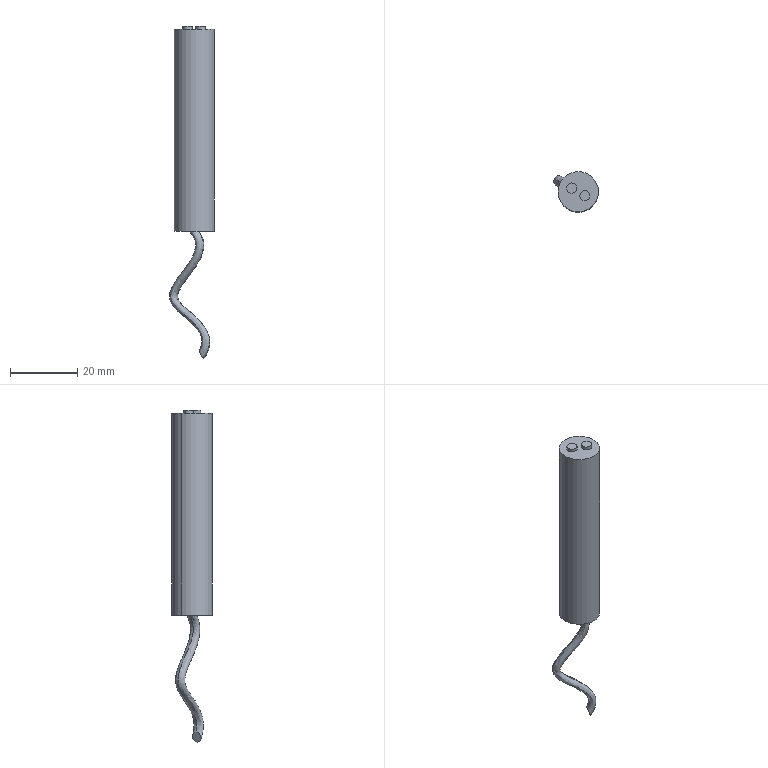Component | SolidWorks | 04_12PhotoelectricSwitch-3 | 1 solid | 13 faces | box 13.38 x 12 x 98.73 mm | volume 7034 mm3 | cylinder 6 | plane 5 | spline 2 | commonest cylinder face diameters 3 x4 12 x2
STEP:
#1=CARTESIAN_POINT('',(3.235,-4.292,15.551));
#2=VERTEX_POINT('',#1);
#3=CARTESIAN_POINT('',(3.133,-4.233,15.551));
#4=VERTEX_POINT('',#3);
#5=CARTESIAN_POINT('',(3.184,-4.263,15.551));
#6=DIRECTION('',(-0.,0.,1.));
#7=DIRECTION('',(-0.8652,0.5014,0.));
#8=AXIS2_PLACEMENT_3D('',#5,#6,#7);
#9=CIRCLE('',#8,0.05906);
#10=EDGE_CURVE('',#2,#4,#9,.T.);
#11=ORIENTED_EDGE('',*,*,#10,.F.);
#12=CARTESIAN_POINT('',(3.235,-4.292,15.512));
#13=VERTEX_POINT('',#12);
#14=CARTESIAN_POINT('',(3.235,-4.292,15.551));
#15=DIRECTION('',(0.,-0.,-1.));
#16=VECTOR('',#15,39.37);
#17=LINE('',#14,#16);
#18=EDGE_CURVE('',#2,#13,#17,.T.);
#19=ORIENTED_EDGE('',*,*,#18,.T.);
#20=CARTESIAN_POINT('',(3.133,-4.233,15.512));
#21=VERTEX_POINT('',#20);
#22=CARTESIAN_POINT('',(3.184,-4.263,15.512));
#23=DIRECTION('',(-0.,0.,1.));
#24=DIRECTION('',(-0.8652,0.5014,0.));
#25=AXIS2_PLACEMENT_3D('',#22,#23,#24);
#26=CIRCLE('',#25,0.05906);
#27=EDGE_CURVE('',#13,#21,#26,.T.);
#28=ORIENTED_EDGE('',*,*,#27,.T.);
#29=CARTESIAN_POINT('',(3.133,-4.233,15.551));
#30=DIRECTION('',(0.,-0.,-1.));
#31=VECTOR('',#30,39.37);
#32=LINE('',#29,#31);
#33=EDGE_CURVE('',#4,#21,#32,.T.);
#34=ORIENTED_EDGE('',*,*,#33,.F.);
#35=EDGE_LOOP('',(#11,#19,#28,#34));
#36=FACE_OUTER_BOUND('',#35,.T.);
#37=CARTESIAN_POINT('',(3.184,-4.263,15.551));
#38=DIRECTION('',(0.,-0.,-1.));
#39=DIRECTION('',(-0.8652,0.5014,0.));
#40=AXIS2_PLACEMENT_3D('',#37,#38,#39);
#41=CYLINDRICAL_SURFACE('',#40,0.05906);
#42=ADVANCED_FACE('',(#36),#41,.T.);
#43=CARTESIAN_POINT('',(3.082,-4.203,15.551));
#44=VERTEX_POINT('',#43);
#45=CARTESIAN_POINT('',(2.98,-4.144,15.551));
#46=VERTEX_POINT('',#45);
#47=CARTESIAN_POINT('',(3.031,-4.174,15.551));
#48=DIRECTION('',(-0.,0.,1.));
#49=DIRECTION('',(0.8652,-0.5014,0.));
#50=AXIS2_PLACEMENT_3D('',#47,#48,#49);
#51=CIRCLE('',#50,0.05906);
#52=EDGE_CURVE('',#44,#46,#51,.T.);
#53=ORIENTED_EDGE('',*,*,#52,.F.);
#54=CARTESIAN_POINT('',(3.082,-4.203,15.512));
#55=VERTEX_POINT('',#54);
#56=CARTESIAN_POINT('',(3.082,-4.203,15.551));
#57=DIRECTION('',(0.,-0.,-1.));
#58=VECTOR('',#57,39.37);
#59=LINE('',#56,#58);
#60=EDGE_CURVE('',#44,#55,#59,.T.);
#61=ORIENTED_EDGE('',*,*,#60,.T.);
#62=CARTESIAN_POINT('',(2.98,-4.144,15.512));
#63=VERTEX_POINT('',#62);
#64=CARTESIAN_POINT('',(3.031,-4.174,15.512));
#65=DIRECTION('',(-0.,0.,1.));
#66=DIRECTION('',(0.8652,-0.5014,0.));
#67=AXIS2_PLACEMENT_3D('',#64,#65,#66);
#68=CIRCLE('',#67,0.05906);
#69=EDGE_CURVE('',#55,#63,#68,.T.);
#70=ORIENTED_EDGE('',*,*,#69,.T.);
#71=CARTESIAN_POINT('',(2.98,-4.144,15.551));
#72=DIRECTION('',(0.,-0.,-1.));
#73=VECTOR('',#72,39.37);
#74=LINE('',#71,#73);
#75=EDGE_CURVE('',#46,#63,#74,.T.);
#76=ORIENTED_EDGE('',*,*,#75,.F.);
#77=EDGE_LOOP('',(#53,#61,#70,#76));
#78=FACE_OUTER_BOUND('',#77,.T.);
#79=CARTESIAN_POINT('',(3.031,-4.174,15.551));
#80=DIRECTION('',(0.,-0.,-1.));
#81=DIRECTION('',(-0.8652,0.5014,0.));
#82=AXIS2_PLACEMENT_3D('',#79,#80,#81);
#83=CYLINDRICAL_SURFACE('',#82,0.05906);
#84=ADVANCED_FACE('',(#78),#83,.T.);
#85=CARTESIAN_POINT('',(3.056,-4.189,13.15));
#86=VERTEX_POINT('',#85);
#87=CARTESIAN_POINT('',(3.158,-4.248,13.15));
#88=VERTEX_POINT('',#87);
#89=CARTESIAN_POINT('',(3.107,-4.218,13.15));
#90=DIRECTION('',(0.,-0.,-1.));
#91=DIRECTION('',(-0.8652,0.5014,0.));
#92=AXIS2_PLACEMENT_3D('',#89,#90,#91);
#93=CIRCLE('',#92,0.05906);
#94=EDGE_CURVE('',#86,#88,#93,.T.);
#95=ORIENTED_EDGE('',*,*,#94,.T.);
#96=CARTESIAN_POINT('',(3.218,-4.282,11.664));
#97=VERTEX_POINT('',#96);
#98=CARTESIAN_POINT('',(3.158,-4.248,13.15));
#99=CARTESIAN_POINT('',(3.169,-4.254,13.132));
#100=CARTESIAN_POINT('',(3.188,-4.265,13.098));
#101=CARTESIAN_POINT('',(3.204,-4.275,13.044));
#102=CARTESIAN_POINT('',(3.211,-4.278,12.992));
#103=CARTESIAN_POINT('',(3.208,-4.276,12.941));
#104=CARTESIAN_POINT('',(3.195,-4.269,12.882));
#105=CARTESIAN_POINT('',(3.169,-4.254,12.818));
#106=CARTESIAN_POINT('',(3.13,-4.232,12.749));
#107=CARTESIAN_POINT('',(3.05,-4.185,12.633));
#108=CARTESIAN_POINT('',(2.964,-4.135,12.532));
#109=CARTESIAN_POINT('',(2.917,-4.108,12.446));
#110=CARTESIAN_POINT('',(2.904,-4.101,12.412));
#111=CARTESIAN_POINT('',(2.899,-4.097,12.381));
#112=CARTESIAN_POINT('',(2.902,-4.099,12.355));
#113=CARTESIAN_POINT('',(2.91,-4.104,12.343));
#114=CARTESIAN_POINT('',(2.918,-4.108,12.332));
#115=CARTESIAN_POINT('',(2.927,-4.114,12.323));
#116=CARTESIAN_POINT('',(2.943,-4.123,12.305));
#117=CARTESIAN_POINT('',(2.964,-4.135,12.284));
#118=CARTESIAN_POINT('',(3.021,-4.168,12.231));
#119=CARTESIAN_POINT('',(3.112,-4.221,12.16));
#120=CARTESIAN_POINT('',(3.201,-4.272,12.066));
#121=CARTESIAN_POINT('',(3.246,-4.299,12.001));
#122=CARTESIAN_POINT('',(3.272,-4.314,11.939));
#123=CARTESIAN_POINT('',(3.281,-4.319,11.884));
#124=CARTESIAN_POINT('',(3.282,-4.32,11.841));
#125=CARTESIAN_POINT('',(3.276,-4.316,11.797));
#126=CARTESIAN_POINT('',(3.264,-4.309,11.753));
#127=CARTESIAN_POINT('',(3.245,-4.298,11.709));
#128=CARTESIAN_POINT('',(3.228,-4.288,11.679));
#129=CARTESIAN_POINT('',(3.218,-4.282,11.664));
#130=B_SPLINE_CURVE_WITH_KNOTS('',3,(#98,#99,#100,#101,#102,#103,#104,#105,#106,#107,#108,#109,#110,#111,#112,#113,#114,#115,#116,#117,#118,#119,#120,#121,#122,#123,#124,#125,#126,#127,#128,#129),.UNSPECIFIED.,.F.,.F.,(4,1,1,1,1,1,1,1,1,1,1,1,1,1,1,1,1,1,1,1,1,1,1,1,1,1,1,1,1,4),(0.,0.025,0.05,0.075,0.1,0.125,0.1667,0.2083,0.25,0.39,0.4175,0.445,0.4725,0.5,0.525,0.5257,0.55,0.575,0.6,0.625,0.75,0.7917,0.8333,0.875,0.8958,0.9167,0.9375,0.9583,0.9792,1.),.UNSPECIFIED.);
#131=EDGE_CURVE('',#88,#97,#130,.T.);
#132=ORIENTED_EDGE('',*,*,#131,.T.);
#133=CARTESIAN_POINT('',(3.188,-4.265,11.777));
#134=VERTEX_POINT('',#133);
#135=CARTESIAN_POINT('',(3.203,-4.274,11.72));
#136=DIRECTION('',(0.8274,-0.4795,0.2923));
#137=DIRECTION('',(0.2529,-0.1466,-0.9563));
#138=AXIS2_PLACEMENT_3D('',#135,#136,#137);
#139=CIRCLE('',#138,0.05906);
#140=EDGE_CURVE('',#97,#134,#139,.T.);
#141=ORIENTED_EDGE('',*,*,#140,.T.);
#142=CARTESIAN_POINT('',(3.056,-4.189,13.15));
#143=CARTESIAN_POINT('',(3.067,-4.195,13.138));
#144=CARTESIAN_POINT('',(3.086,-4.206,13.116));
#145=CARTESIAN_POINT('',(3.108,-4.218,13.084));
#146=CARTESIAN_POINT('',(3.123,-4.227,13.053));
#147=CARTESIAN_POINT('',(3.132,-4.232,13.021));
#148=CARTESIAN_POINT('',(3.136,-4.235,12.979));
#149=CARTESIAN_POINT('',(3.128,-4.23,12.927));
#150=CARTESIAN_POINT('',(3.104,-4.216,12.864));
#151=CARTESIAN_POINT('',(3.039,-4.179,12.751));
#152=CARTESIAN_POINT('',(2.955,-4.13,12.65));
#153=CARTESIAN_POINT('',(2.892,-4.093,12.56));
#154=CARTESIAN_POINT('',(2.868,-4.079,12.523));
#155=CARTESIAN_POINT('',(2.847,-4.068,12.483));
#156=CARTESIAN_POINT('',(2.832,-4.059,12.443));
#157=CARTESIAN_POINT('',(2.826,-4.055,12.412));
#158=CARTESIAN_POINT('',(2.825,-4.055,12.383));
#159=CARTESIAN_POINT('',(2.827,-4.056,12.354));
#160=CARTESIAN_POINT('',(2.841,-4.064,12.316));
#161=CARTESIAN_POINT('',(2.861,-4.076,12.28));
#162=CARTESIAN_POINT('',(2.92,-4.11,12.204));
#163=CARTESIAN_POINT('',(3.012,-4.163,12.133));
#164=CARTESIAN_POINT('',(3.099,-4.213,12.055));
#165=CARTESIAN_POINT('',(3.143,-4.239,12.008));
#166=CARTESIAN_POINT('',(3.172,-4.256,11.969));
#167=CARTESIAN_POINT('',(3.189,-4.266,11.937));
#168=CARTESIAN_POINT('',(3.199,-4.272,11.911));
#169=CARTESIAN_POINT('',(3.206,-4.275,11.883));
#170=CARTESIAN_POINT('',(3.207,-4.276,11.852));
#171=CARTESIAN_POINT('',(3.202,-4.273,11.817));
#172=CARTESIAN_POINT('',(3.194,-4.268,11.79));
#173=CARTESIAN_POINT('',(3.188,-4.265,11.777));
#174=B_SPLINE_CURVE_WITH_KNOTS('',3,(#142,#143,#144,#145,#146,#147,#148,#149,#150,#151,#152,#153,#154,#155,#156,#157,#158,#159,#160,#161,#162,#163,#164,#165,#166,#167,#168,#169,#170,#171,#172,#173),.UNSPECIFIED.,.F.,.F.,(4,1,1,1,1,1,1,1,1,1,1,1,1,1,1,1,1,1,1,1,1,1,1,1,1,1,1,1,1,4),(0.,0.025,0.05,0.075,0.1,0.125,0.1667,0.2083,0.25,0.39,0.4175,0.445,0.4725,0.5,0.525,0.5257,0.55,0.575,0.6,0.625,0.75,0.7917,0.8333,0.875,0.8958,0.9167,0.9375,0.9583,0.9792,1.),.UNSPECIFIED.);
#175=EDGE_CURVE('',#86,#134,#174,.T.);
#176=ORIENTED_EDGE('',*,*,#175,.F.);
#177=EDGE_LOOP('',(#95,#132,#141,#176));
#178=FACE_OUTER_BOUND('',#177,.T.);
#179=CARTESIAN_POINT('',(3.056,-4.189,13.15));
#180=CARTESIAN_POINT('',(3.067,-4.195,13.138));
#181=CARTESIAN_POINT('',(3.086,-4.206,13.116));
#182=CARTESIAN_POINT('',(3.108,-4.218,13.084));
#183=CARTESIAN_POINT('',(3.123,-4.227,13.053));
#184=CARTESIAN_POINT('',(3.132,-4.232,13.021));
#185=CARTESIAN_POINT('',(3.136,-4.235,12.979));
#186=CARTESIAN_POINT('',(3.128,-4.23,12.927));
#187=CARTESIAN_POINT('',(3.104,-4.216,12.864));
#188=CARTESIAN_POINT('',(3.039,-4.179,12.751));
#189=CARTESIAN_POINT('',(2.955,-4.13,12.65));
#190=CARTESIAN_POINT('',(2.892,-4.093,12.56));
#191=CARTESIAN_POINT('',(2.868,-4.079,12.523));
#192=CARTESIAN_POINT('',(2.847,-4.068,12.483));
#193=CARTESIAN_POINT('',(2.832,-4.059,12.443));
#194=CARTESIAN_POINT('',(2.826,-4.055,12.412));
#195=CARTESIAN_POINT('',(2.825,-4.055,12.383));
#196=CARTESIAN_POINT('',(2.827,-4.056,12.354));
#197=CARTESIAN_POINT('',(2.841,-4.064,12.316));
#198=CARTESIAN_POINT('',(2.861,-4.076,12.28));
#199=CARTESIAN_POINT('',(2.92,-4.11,12.204));
#200=CARTESIAN_POINT('',(3.012,-4.163,12.133));
#201=CARTESIAN_POINT('',(3.099,-4.213,12.055));
#202=CARTESIAN_POINT('',(3.143,-4.239,12.008));
#203=CARTESIAN_POINT('',(3.172,-4.256,11.969));
#204=CARTESIAN_POINT('',(3.189,-4.266,11.937));
#205=CARTESIAN_POINT('',(3.199,-4.272,11.911));
#206=CARTESIAN_POINT('',(3.206,-4.275,11.883));
#207=CARTESIAN_POINT('',(3.207,-4.276,11.852));
#208=CARTESIAN_POINT('',(3.202,-4.273,11.817));
#209=CARTESIAN_POINT('',(3.194,-4.268,11.79));
#210=CARTESIAN_POINT('',(3.188,-4.265,11.777));
#211=CARTESIAN_POINT('',(3.115,-4.086,13.15));
#212=CARTESIAN_POINT('',(3.127,-4.093,13.138));
#213=CARTESIAN_POINT('',(3.146,-4.104,13.116));
#214=CARTESIAN_POINT('',(3.167,-4.116,13.084));
#215=CARTESIAN_POINT('',(3.182,-4.125,13.053));
#216=CARTESIAN_POINT('',(3.191,-4.13,13.021));
#217=CARTESIAN_POINT('',(3.195,-4.132,12.979));
#218=CARTESIAN_POINT('',(3.187,-4.128,12.927));
#219=CARTESIAN_POINT('',(3.163,-4.114,12.864));
#220=CARTESIAN_POINT('',(3.099,-4.077,12.751));
#221=CARTESIAN_POINT('',(3.014,-4.028,12.65));
#222=CARTESIAN_POINT('',(2.951,-3.991,12.56));
#223=CARTESIAN_POINT('',(2.927,-3.977,12.523));
#224=CARTESIAN_POINT('',(2.907,-3.965,12.483));
#225=CARTESIAN_POINT('',(2.891,-3.957,12.443));
#226=CARTESIAN_POINT('',(2.886,-3.953,12.412));
#227=CARTESIAN_POINT('',(2.884,-3.952,12.383));
#228=CARTESIAN_POINT('',(2.887,-3.954,12.354));
#229=CARTESIAN_POINT('',(2.9,-3.962,12.316));
#230=CARTESIAN_POINT('',(2.921,-3.973,12.28));
#231=CARTESIAN_POINT('',(2.98,-4.008,12.204));
#232=CARTESIAN_POINT('',(3.071,-4.061,12.133));
#233=CARTESIAN_POINT('',(3.158,-4.111,12.055));
#234=CARTESIAN_POINT('',(3.202,-4.137,12.008));
#235=CARTESIAN_POINT('',(3.231,-4.154,11.969));
#236=CARTESIAN_POINT('',(3.249,-4.164,11.937));
#237=CARTESIAN_POINT('',(3.259,-4.169,11.911));
#238=CARTESIAN_POINT('',(3.265,-4.173,11.883));
#239=CARTESIAN_POINT('',(3.266,-4.174,11.852));
#240=CARTESIAN_POINT('',(3.261,-4.171,11.817));
#241=CARTESIAN_POINT('',(3.253,-4.166,11.79));
#242=CARTESIAN_POINT('',(3.247,-4.163,11.777));
#243=CARTESIAN_POINT('',(3.218,-4.146,13.15));
#244=CARTESIAN_POINT('',(3.229,-4.152,13.132));
#245=CARTESIAN_POINT('',(3.247,-4.163,13.098));
#246=CARTESIAN_POINT('',(3.264,-4.172,13.044));
#247=CARTESIAN_POINT('',(3.27,-4.176,12.992));
#248=CARTESIAN_POINT('',(3.267,-4.174,12.941));
#249=CARTESIAN_POINT('',(3.254,-4.167,12.882));
#250=CARTESIAN_POINT('',(3.228,-4.152,12.818));
#251=CARTESIAN_POINT('',(3.189,-4.129,12.749));
#252=CARTESIAN_POINT('',(3.109,-4.083,12.633));
#253=CARTESIAN_POINT('',(3.023,-4.033,12.532));
#254=CARTESIAN_POINT('',(2.977,-4.006,12.446));
#255=CARTESIAN_POINT('',(2.963,-3.998,12.412));
#256=CARTESIAN_POINT('',(2.958,-3.995,12.381));
#257=CARTESIAN_POINT('',(2.961,-3.997,12.355));
#258=CARTESIAN_POINT('',(2.969,-4.001,12.343));
#259=CARTESIAN_POINT('',(2.977,-4.006,12.332));
#260=CARTESIAN_POINT('',(2.986,-4.011,12.323));
#261=CARTESIAN_POINT('',(3.002,-4.021,12.305));
#262=CARTESIAN_POINT('',(3.023,-4.033,12.284));
#263=CARTESIAN_POINT('',(3.08,-4.066,12.231));
#264=CARTESIAN_POINT('',(3.171,-4.119,12.16));
#265=CARTESIAN_POINT('',(3.26,-4.17,12.066));
#266=CARTESIAN_POINT('',(3.305,-4.196,12.001));
#267=CARTESIAN_POINT('',(3.331,-4.211,11.939));
#268=CARTESIAN_POINT('',(3.341,-4.217,11.884));
#269=CARTESIAN_POINT('',(3.341,-4.217,11.841));
#270=CARTESIAN_POINT('',(3.335,-4.214,11.797));
#271=CARTESIAN_POINT('',(3.323,-4.207,11.753));
#272=CARTESIAN_POINT('',(3.304,-4.196,11.709));
#273=CARTESIAN_POINT('',(3.287,-4.186,11.679));
#274=CARTESIAN_POINT('',(3.277,-4.18,11.664));
#275=CARTESIAN_POINT('',(3.158,-4.248,13.15));
#276=CARTESIAN_POINT('',(3.169,-4.254,13.132));
#277=CARTESIAN_POINT('',(3.188,-4.265,13.098));
#278=CARTESIAN_POINT('',(3.204,-4.275,13.044));
#279=CARTESIAN_POINT('',(3.211,-4.278,12.992));
#280=CARTESIAN_POINT('',(3.208,-4.276,12.941));
#281=CARTESIAN_POINT('',(3.195,-4.269,12.882));
#282=CARTESIAN_POINT('',(3.169,-4.254,12.818));
#283=CARTESIAN_POINT('',(3.13,-4.232,12.749));
#284=CARTESIAN_POINT('',(3.05,-4.185,12.633));
#285=CARTESIAN_POINT('',(2.964,-4.135,12.532));
#286=CARTESIAN_POINT('',(2.917,-4.108,12.446));
#287=CARTESIAN_POINT('',(2.904,-4.101,12.412));
#288=CARTESIAN_POINT('',(2.899,-4.097,12.381));
#289=CARTESIAN_POINT('',(2.902,-4.099,12.355));
#290=CARTESIAN_POINT('',(2.91,-4.104,12.343));
#291=CARTESIAN_POINT('',(2.918,-4.108,12.332));
#292=CARTESIAN_POINT('',(2.927,-4.114,12.323));
#293=CARTESIAN_POINT('',(2.943,-4.123,12.305));
#294=CARTESIAN_POINT('',(2.964,-4.135,12.284));
#295=CARTESIAN_POINT('',(3.021,-4.168,12.231));
#296=CARTESIAN_POINT('',(3.112,-4.221,12.16));
#297=CARTESIAN_POINT('',(3.201,-4.272,12.066));
#298=CARTESIAN_POINT('',(3.246,-4.299,12.001));
#299=CARTESIAN_POINT('',(3.272,-4.314,11.939));
#300=CARTESIAN_POINT('',(3.281,-4.319,11.884));
#301=CARTESIAN_POINT('',(3.282,-4.32,11.841));
#302=CARTESIAN_POINT('',(3.276,-4.316,11.797));
#303=CARTESIAN_POINT('',(3.264,-4.309,11.753));
#304=CARTESIAN_POINT('',(3.245,-4.298,11.709));
#305=CARTESIAN_POINT('',(3.228,-4.288,11.679));
#306=CARTESIAN_POINT('',(3.218,-4.282,11.664));
#307=CARTESIAN_POINT('',(3.099,-4.35,13.15));
#308=CARTESIAN_POINT('',(3.11,-4.356,13.132));
#309=CARTESIAN_POINT('',(3.129,-4.367,13.098));
#310=CARTESIAN_POINT('',(3.145,-4.377,13.044));
#311=CARTESIAN_POINT('',(3.151,-4.38,12.992));
#312=CARTESIAN_POINT('',(3.148,-4.379,12.941));
#313=CARTESIAN_POINT('',(3.136,-4.371,12.882));
#314=CARTESIAN_POINT('',(3.11,-4.356,12.818));
#315=CARTESIAN_POINT('',(3.071,-4.334,12.749));
#316=CARTESIAN_POINT('',(2.991,-4.287,12.633));
#317=CARTESIAN_POINT('',(2.905,-4.237,12.532));
#318=CARTESIAN_POINT('',(2.858,-4.21,12.446));
#319=CARTESIAN_POINT('',(2.845,-4.203,12.412));
#320=CARTESIAN_POINT('',(2.84,-4.2,12.381));
#321=CARTESIAN_POINT('',(2.843,-4.202,12.355));
#322=CARTESIAN_POINT('',(2.85,-4.206,12.343));
#323=CARTESIAN_POINT('',(2.858,-4.211,12.332));
#324=CARTESIAN_POINT('',(2.868,-4.216,12.323));
#325=CARTESIAN_POINT('',(2.884,-4.225,12.305));
#326=CARTESIAN_POINT('',(2.904,-4.237,12.284));
#327=CARTESIAN_POINT('',(2.962,-4.27,12.231));
#328=CARTESIAN_POINT('',(3.052,-4.323,12.16));
#329=CARTESIAN_POINT('',(3.141,-4.375,12.066));
#330=CARTESIAN_POINT('',(3.187,-4.401,12.001));
#331=CARTESIAN_POINT('',(3.212,-4.416,11.939));
#332=CARTESIAN_POINT('',(3.222,-4.421,11.884));
#333=CARTESIAN_POINT('',(3.223,-4.422,11.841));
#334=CARTESIAN_POINT('',(3.217,-4.418,11.797));
#335=CARTESIAN_POINT('',(3.204,-4.411,11.753));
#336=CARTESIAN_POINT('',(3.185,-4.4,11.709));
#337=CARTESIAN_POINT('',(3.169,-4.39,11.679));
#338=CARTESIAN_POINT('',(3.159,-4.385,11.664));
#339=CARTESIAN_POINT('',(2.997,-4.291,13.15));
#340=CARTESIAN_POINT('',(3.008,-4.297,13.138));
#341=CARTESIAN_POINT('',(3.027,-4.308,13.116));
#342=CARTESIAN_POINT('',(3.048,-4.321,13.084));
#343=CARTESIAN_POINT('',(3.063,-4.329,13.053));
#344=CARTESIAN_POINT('',(3.072,-4.335,13.021));
#345=CARTESIAN_POINT('',(3.076,-4.337,12.979));
#346=CARTESIAN_POINT('',(3.069,-4.332,12.927));
#347=CARTESIAN_POINT('',(3.044,-4.318,12.864));
#348=CARTESIAN_POINT('',(2.98,-4.281,12.751));
#349=CARTESIAN_POINT('',(2.895,-4.232,12.65));
#350=CARTESIAN_POINT('',(2.833,-4.196,12.56));
#351=CARTESIAN_POINT('',(2.809,-4.182,12.523));
#352=CARTESIAN_POINT('',(2.788,-4.17,12.483));
#353=CARTESIAN_POINT('',(2.773,-4.161,12.443));
#354=CARTESIAN_POINT('',(2.767,-4.158,12.412));
#355=CARTESIAN_POINT('',(2.766,-4.157,12.383));
#356=CARTESIAN_POINT('',(2.768,-4.158,12.354));
#357=CARTESIAN_POINT('',(2.782,-4.166,12.316));
#358=CARTESIAN_POINT('',(2.802,-4.178,12.28));
#359=CARTESIAN_POINT('',(2.861,-4.212,12.204));
#360=CARTESIAN_POINT('',(2.953,-4.265,12.133));
#361=CARTESIAN_POINT('',(3.039,-4.315,12.055));
#362=CARTESIAN_POINT('',(3.084,-4.341,12.008));
#363=CARTESIAN_POINT('',(3.113,-4.358,11.969));
#364=CARTESIAN_POINT('',(3.13,-4.368,11.937));
#365=CARTESIAN_POINT('',(3.14,-4.374,11.911));
#366=CARTESIAN_POINT('',(3.146,-4.377,11.883));
#367=CARTESIAN_POINT('',(3.148,-4.378,11.852));
#368=CARTESIAN_POINT('',(3.143,-4.375,11.817));
#369=CARTESIAN_POINT('',(3.135,-4.371,11.79));
#370=CARTESIAN_POINT('',(3.129,-4.367,11.777));
#371=CARTESIAN_POINT('',(3.056,-4.189,13.15));
#372=CARTESIAN_POINT('',(3.067,-4.195,13.138));
#373=CARTESIAN_POINT('',(3.086,-4.206,13.116));
#374=CARTESIAN_POINT('',(3.108,-4.218,13.084));
#375=CARTESIAN_POINT('',(3.123,-4.227,13.053));
#376=CARTESIAN_POINT('',(3.132,-4.232,13.021));
#377=CARTESIAN_POINT('',(3.136,-4.235,12.979));
#378=CARTESIAN_POINT('',(3.128,-4.23,12.927));
#379=CARTESIAN_POINT('',(3.104,-4.216,12.864));
#380=CARTESIAN_POINT('',(3.039,-4.179,12.751));
#381=CARTESIAN_POINT('',(2.955,-4.13,12.65));
#382=CARTESIAN_POINT('',(2.892,-4.093,12.56));
#383=CARTESIAN_POINT('',(2.868,-4.079,12.523));
#384=CARTESIAN_POINT('',(2.847,-4.068,12.483));
#385=CARTESIAN_POINT('',(2.832,-4.059,12.443));
#386=CARTESIAN_POINT('',(2.826,-4.055,12.412));
#387=CARTESIAN_POINT('',(2.825,-4.055,12.383));
#388=CARTESIAN_POINT('',(2.827,-4.056,12.354));
#389=CARTESIAN_POINT('',(2.841,-4.064,12.316));
#390=CARTESIAN_POINT('',(2.861,-4.076,12.28));
#391=CARTESIAN_POINT('',(2.92,-4.11,12.204));
#392=CARTESIAN_POINT('',(3.012,-4.163,12.133));
#393=CARTESIAN_POINT('',(3.099,-4.213,12.055));
#394=CARTESIAN_POINT('',(3.143,-4.239,12.008));
#395=CARTESIAN_POINT('',(3.172,-4.256,11.969));
#396=CARTESIAN_POINT('',(3.189,-4.266,11.937));
#397=CARTESIAN_POINT('',(3.199,-4.272,11.911));
#398=CARTESIAN_POINT('',(3.206,-4.275,11.883));
#399=CARTESIAN_POINT('',(3.207,-4.276,11.852));
#400=CARTESIAN_POINT('',(3.202,-4.273,11.817));
#401=CARTESIAN_POINT('',(3.194,-4.268,11.79));
#402=CARTESIAN_POINT('',(3.188,-4.265,11.777));
#403=(BOUNDED_SURFACE()B_SPLINE_SURFACE(3,3,((#179,#180,#181,#182,#183,#184,#185,#186,#187,#188,#189,#190,#191,#192,#193,#194,#195,#196,#197,#198,#199,#200,#201,#202,#203,#204,#205,#206,#207,#208,#209,#210),(#211,#212,#213,#214,#215,#216,#217,#218,#219,#220,#221,#222,#223,#224,#225,#226,#227,#228,#229,#230,#231,#232,#233,#234,#235,#236,#237,#238,#239,#240,#241,#242),(#243,#244,#245,#246,#247,#248,#249,#250,#251,#252,#253,#254,#255,#256,#257,#258,#259,#260,#261,#262,#263,#264,#265,#266,#267,#268,#269,#270,#271,#272,#273,#274),(#275,#276,#277,#278,#279,#280,#281,#282,#283,#284,#285,#286,#287,#288,#289,#290,#291,#292,#293,#294,#295,#296,#297,#298,#299,#300,#301,#302,#303,#304,#305,#306),(#307,#308,#309,#310,#311,#312,#313,#314,#315,#316,#317,#318,#319,#320,#321,#322,#323,#324,#325,#326,#327,#328,#329,#330,#331,#332,#333,#334,#335,#336,#337,#338),(#339,#340,#341,#342,#343,#344,#345,#346,#347,#348,#349,#350,#351,#352,#353,#354,#355,#356,#357,#358,#359,#360,#361,#362,#363,#364,#365,#366,#367,#368,#369,#370),(#371,#372,#373,#374,#375,#376,#377,#378,#379,#380,#381,#382,#383,#384,#385,#386,#387,#388,#389,#390,#391,#392,#393,#394,#395,#396,#397,#398,#399,#400,#401,#402)),.UNSPECIFIED.,.T.,.F.,.F.)B_SPLINE_SURFACE_WITH_KNOTS((4,3,4),(4,1,1,1,1,1,1,1,1,1,1,1,1,1,1,1,1,1,1,1,1,1,1,1,1,1,1,1,1,4),(0.,0.5,1.),(0.,0.025,0.05,0.075,0.1,0.125,0.1667,0.2083,0.25,0.39,0.4175,0.445,0.4725,0.5,0.525,0.5257,0.55,0.575,0.6,0.625,0.75,0.7917,0.8333,0.875,0.8958,0.9167,0.9375,0.9583,0.9792,1.),.UNSPECIFIED.)GEOMETRIC_REPRESENTATION_ITEM()RATIONAL_B_SPLINE_SURFACE(((1.,1.,1.,1.,1.,1.,1.,1.,1.,1.,1.,1.,1.,1.,1.,1.,1.,1.,1.,1.,1.,1.,1.,1.,1.,1.,1.,1.,1.,1.,1.,1.),(0.3333,0.3333,0.3333,0.3333,0.3333,0.3333,0.3333,0.3333,0.3333,0.3333,0.3333,0.3333,0.3333,0.3333,0.3333,0.3333,0.3333,0.3333,0.3333,0.3333,0.3333,0.3333,0.3333,0.3333,0.3333,0.3333,0.3333,0.3333,0.3333,0.3333,0.3333,0.3333),(0.3333,0.3333,0.3333,0.3333,0.3333,0.3333,0.3333,0.3333,0.3333,0.3333,0.3333,0.3333,0.3333,0.3333,0.3333,0.3333,0.3333,0.3333,0.3333,0.3333,0.3333,0.3333,0.3333,0.3333,0.3333,0.3333,0.3333,0.3333,0.3333,0.3333,0.3333,0.3333),(1.,1.,1.,1.,1.,1.,1.,1.,1.,1.,1.,1.,1.,1.,1.,1.,1.,1.,1.,1.,1.,1.,1.,1.,1.,1.,1.,1.,1.,1.,1.,1.),(0.3333,0.3333,0.3333,0.3333,0.3333,0.3333,0.3333,0.3333,0.3333,0.3333,0.3333,0.3333,0.3333,0.3333,0.3333,0.3333,0.3333,0.3333,0.3333,0.3333,0.3333,0.3333,0.3333,0.3333,0.3333,0.3333,0.3333,0.3333,0.3333,0.3333,0.3333,0.3333),(0.3333,0.3333,0.3333,0.3333,0.3333,0.3333,0.3333,0.3333,0.3333,0.3333,0.3333,0.3333,0.3333,0.3333,0.3333,0.3333,0.3333,0.3333,0.3333,0.3333,0.3333,0.3333,0.3333,0.3333,0.3333,0.3333,0.3333,0.3333,0.3333,0.3333,0.3333,0.3333),(1.,1.,1.,1.,1.,1.,1.,1.,1.,1.,1.,1.,1.,1.,1.,1.,1.,1.,1.,1.,1.,1.,1.,1.,1.,1.,1.,1.,1.,1.,1.,1.)))REPRESENTATION_ITEM('')SURFACE());
#404=ADVANCED_FACE('',(#178),#403,.T.);
#405=CARTESIAN_POINT('',(3.312,-4.337,15.512));
#406=VERTEX_POINT('',#405);
#407=CARTESIAN_POINT('',(2.903,-4.1,15.512));
#408=VERTEX_POINT('',#407);
#409=CARTESIAN_POINT('',(3.107,-4.218,15.512));
#410=DIRECTION('',(-0.,0.,1.));
#411=DIRECTION('',(0.8652,-0.5014,0.));
#412=AXIS2_PLACEMENT_3D('',#409,#410,#411);
#413=CIRCLE('',#412,0.2362);
#414=EDGE_CURVE('',#406,#408,#413,.T.);
#415=ORIENTED_EDGE('',*,*,#414,.F.);
#416=CARTESIAN_POINT('',(3.312,-4.337,13.15));
#417=VERTEX_POINT('',#416);
#418=CARTESIAN_POINT('',(3.312,-4.337,15.512));
#419=DIRECTION('',(0.,-0.,-1.));
#420=VECTOR('',#419,39.37);
#421=LINE('',#418,#420);
#422=EDGE_CURVE('',#406,#417,#421,.T.);
#423=ORIENTED_EDGE('',*,*,#422,.T.);
#424=CARTESIAN_POINT('',(2.903,-4.1,13.15));
#425=VERTEX_POINT('',#424);
#426=CARTESIAN_POINT('',(3.107,-4.218,13.15));
#427=DIRECTION('',(-0.,0.,1.));
#428=DIRECTION('',(0.8652,-0.5014,0.));
#429=AXIS2_PLACEMENT_3D('',#426,#427,#428);
#430=CIRCLE('',#429,0.2362);
#431=EDGE_CURVE('',#417,#425,#430,.T.);
#432=ORIENTED_EDGE('',*,*,#431,.T.);
#433=CARTESIAN_POINT('',(2.903,-4.1,15.512));
#434=DIRECTION('',(0.,-0.,-1.));
#435=VECTOR('',#434,39.37);
#436=LINE('',#433,#435);
#437=EDGE_CURVE('',#408,#425,#436,.T.);
#438=ORIENTED_EDGE('',*,*,#437,.F.);
#439=EDGE_LOOP('',(#415,#423,#432,#438));
#440=FACE_OUTER_BOUND('',#439,.T.);
#441=CARTESIAN_POINT('',(3.107,-4.218,15.512));
#442=DIRECTION('',(0.,-0.,-1.));
#443=DIRECTION('',(-0.8652,0.5014,0.));
#444=AXIS2_PLACEMENT_3D('',#441,#442,#443);
#445=CYLINDRICAL_SURFACE('',#444,0.2362);
#446=ADVANCED_FACE('',(#440),#445,.T.);
#447=ORIENTED_EDGE('',*,*,#422,.F.);
#448=CARTESIAN_POINT('',(3.107,-4.218,15.512));
#449=DIRECTION('',(-0.,0.,1.));
#450=DIRECTION('',(0.8652,-0.5014,0.));
#451=AXIS2_PLACEMENT_3D('',#448,#449,#450);
#452=CIRCLE('',#451,0.2362);
#453=EDGE_CURVE('',#408,#406,#452,.T.);
#454=ORIENTED_EDGE('',*,*,#453,.F.);
#455=ORIENTED_EDGE('',*,*,#437,.T.);
#456=CARTESIAN_POINT('',(3.107,-4.218,13.15));
#457=DIRECTION('',(-0.,0.,1.));
#458=DIRECTION('',(0.8652,-0.5014,0.));
#459=AXIS2_PLACEMENT_3D('',#456,#457,#458);
#460=CIRCLE('',#459,0.2362);
#461=EDGE_CURVE('',#425,#417,#460,.T.);
#462=ORIENTED_EDGE('',*,*,#461,.T.);
#463=EDGE_LOOP('',(#447,#454,#455,#462));
#464=FACE_OUTER_BOUND('',#463,.T.);
#465=CARTESIAN_POINT('',(3.107,-4.218,15.512));
#466=DIRECTION('',(0.,-0.,-1.));
#467=DIRECTION('',(-0.8652,0.5014,0.));
#468=AXIS2_PLACEMENT_3D('',#465,#466,#467);
#469=CYLINDRICAL_SURFACE('',#468,0.2362);
#470=ADVANCED_FACE('',(#464),#469,.T.);
#471=CARTESIAN_POINT('',(3.184,-4.263,15.512));
#472=DIRECTION('',(-0.,0.,1.));
#473=DIRECTION('',(-0.8652,0.5014,0.));
#474=AXIS2_PLACEMENT_3D('',#471,#472,#473);
#475=CIRCLE('',#474,0.05906);
#476=EDGE_CURVE('',#21,#13,#475,.T.);
#477=ORIENTED_EDGE('',*,*,#476,.F.);
#478=ORIENTED_EDGE('',*,*,#27,.F.);
#479=EDGE_LOOP('',(#477,#478));
#480=FACE_BOUND('',#479,.T.);
#481=CARTESIAN_POINT('',(3.031,-4.174,15.512));
#482=DIRECTION('',(-0.,0.,1.));
#483=DIRECTION('',(0.8652,-0.5014,0.));
#484=AXIS2_PLACEMENT_3D('',#481,#482,#483);
#485=CIRCLE('',#484,0.05906);
#486=EDGE_CURVE('',#63,#55,#485,.T.);
#487=ORIENTED_EDGE('',*,*,#486,.F.);
#488=ORIENTED_EDGE('',*,*,#69,.F.);
#489=EDGE_LOOP('',(#487,#488));
#490=FACE_BOUND('',#489,.T.);
#491=ORIENTED_EDGE('',*,*,#453,.T.);
#492=ORIENTED_EDGE('',*,*,#414,.T.);
#493=EDGE_LOOP('',(#491,#492));
#494=FACE_OUTER_BOUND('',#493,.T.);
#495=CARTESIAN_POINT('',(3.107,-4.218,15.512));
#496=DIRECTION('',(-0.,0.,1.));
#497=DIRECTION('',(0.8652,-0.5014,0.));
#498=AXIS2_PLACEMENT_3D('',#495,#496,#497);
#499=PLANE('',#498);
#500=ADVANCED_FACE('',(#480,#490,#494),#499,.T.);
#501=ORIENTED_EDGE('',*,*,#94,.F.);
#502=CARTESIAN_POINT('',(3.107,-4.218,13.15));
#503=DIRECTION('',(0.,-0.,-1.));
#504=DIRECTION('',(-0.8652,0.5014,0.));
#505=AXIS2_PLACEMENT_3D('',#502,#503,#504);
#506=CIRCLE('',#505,0.05906);
#507=EDGE_CURVE('',#88,#86,#506,.T.);
#508=ORIENTED_EDGE('',*,*,#507,.F.);
#509=EDGE_LOOP('',(#501,#508));
#510=FACE_BOUND('',#509,.T.);
#511=ORIENTED_EDGE('',*,*,#461,.F.);
#512=ORIENTED_EDGE('',*,*,#431,.F.);
#513=EDGE_LOOP('',(#511,#512));
#514=FACE_OUTER_BOUND('',#513,.T.);
#515=CARTESIAN_POINT('',(3.107,-4.218,13.15));
#516=DIRECTION('',(-0.,0.,1.));
#517=DIRECTION('',(0.8652,-0.5014,0.));
#518=AXIS2_PLACEMENT_3D('',#515,#516,#517);
#519=PLANE('',#518);
#520=ADVANCED_FACE('',(#510,#514),#519,.F.);
#521=CARTESIAN_POINT('',(3.203,-4.274,11.72));
#522=DIRECTION('',(0.8274,-0.4795,0.2923));
#523=DIRECTION('',(0.2529,-0.1466,-0.9563));
#524=AXIS2_PLACEMENT_3D('',#521,#522,#523);
#525=CIRCLE('',#524,0.05906);
#526=EDGE_CURVE('',#134,#97,#525,.T.);
#527=ORIENTED_EDGE('',*,*,#526,.F.);
#528=ORIENTED_EDGE('',*,*,#140,.F.);
#529=EDGE_LOOP('',(#527,#528));
#530=FACE_OUTER_BOUND('',#529,.T.);
#531=CARTESIAN_POINT('',(3.218,-4.282,11.664));
#532=DIRECTION('',(0.8274,-0.4795,0.2923));
#533=DIRECTION('',(0.2529,-0.1466,-0.9563));
#534=AXIS2_PLACEMENT_3D('',#531,#532,#533);
#535=PLANE('',#534);
#536=ADVANCED_FACE('',(#530),#535,.F.);
#537=ORIENTED_EDGE('',*,*,#131,.F.);
#538=ORIENTED_EDGE('',*,*,#507,.T.);
#539=ORIENTED_EDGE('',*,*,#175,.T.);
#540=ORIENTED_EDGE('',*,*,#526,.T.);
#541=EDGE_LOOP('',(#537,#538,#539,#540));
#542=FACE_OUTER_BOUND('',#541,.T.);
#543=CARTESIAN_POINT('',(3.056,-4.189,13.15));
#544=CARTESIAN_POINT('',(3.067,-4.195,13.138));
#545=CARTESIAN_POINT('',(3.086,-4.206,13.116));
#546=CARTESIAN_POINT('',(3.108,-4.218,13.084));
#547=CARTESIAN_POINT('',(3.123,-4.227,13.053));
#548=CARTESIAN_POINT('',(3.132,-4.232,13.021));
#549=CARTESIAN_POINT('',(3.136,-4.235,12.979));
#550=CARTESIAN_POINT('',(3.128,-4.23,12.927));
#551=CARTESIAN_POINT('',(3.104,-4.216,12.864));
#552=CARTESIAN_POINT('',(3.039,-4.179,12.751));
#553=CARTESIAN_POINT('',(2.955,-4.13,12.65));
#554=CARTESIAN_POINT('',(2.892,-4.093,12.56));
#555=CARTESIAN_POINT('',(2.868,-4.079,12.523));
#556=CARTESIAN_POINT('',(2.847,-4.068,12.483));
#557=CARTESIAN_POINT('',(2.832,-4.059,12.443));
#558=CARTESIAN_POINT('',(2.826,-4.055,12.412));
#559=CARTESIAN_POINT('',(2.825,-4.055,12.383));
#560=CARTESIAN_POINT('',(2.827,-4.056,12.354));
#561=CARTESIAN_POINT('',(2.841,-4.064,12.316));
#562=CARTESIAN_POINT('',(2.861,-4.076,12.28));
#563=CARTESIAN_POINT('',(2.92,-4.11,12.204));
#564=CARTESIAN_POINT('',(3.012,-4.163,12.133));
#565=CARTESIAN_POINT('',(3.099,-4.213,12.055));
#566=CARTESIAN_POINT('',(3.143,-4.239,12.008));
#567=CARTESIAN_POINT('',(3.172,-4.256,11.969));
#568=CARTESIAN_POINT('',(3.189,-4.266,11.937));
#569=CARTESIAN_POINT('',(3.199,-4.272,11.911));
#570=CARTESIAN_POINT('',(3.206,-4.275,11.883));
#571=CARTESIAN_POINT('',(3.207,-4.276,11.852));
#572=CARTESIAN_POINT('',(3.202,-4.273,11.817));
#573=CARTESIAN_POINT('',(3.194,-4.268,11.79));
#574=CARTESIAN_POINT('',(3.188,-4.265,11.777));
#575=CARTESIAN_POINT('',(3.115,-4.086,13.15));
#576=CARTESIAN_POINT('',(3.127,-4.093,13.138));
#577=CARTESIAN_POINT('',(3.146,-4.104,13.116));
#578=CARTESIAN_POINT('',(3.167,-4.116,13.084));
#579=CARTESIAN_POINT('',(3.182,-4.125,13.053));
#580=CARTESIAN_POINT('',(3.191,-4.13,13.021));
#581=CARTESIAN_POINT('',(3.195,-4.132,12.979));
#582=CARTESIAN_POINT('',(3.187,-4.128,12.927));
#583=CARTESIAN_POINT('',(3.163,-4.114,12.864));
#584=CARTESIAN_POINT('',(3.099,-4.077,12.751));
#585=CARTESIAN_POINT('',(3.014,-4.028,12.65));
#586=CARTESIAN_POINT('',(2.951,-3.991,12.56));
#587=CARTESIAN_POINT('',(2.927,-3.977,12.523));
#588=CARTESIAN_POINT('',(2.907,-3.965,12.483));
#589=CARTESIAN_POINT('',(2.891,-3.957,12.443));
#590=CARTESIAN_POINT('',(2.886,-3.953,12.412));
#591=CARTESIAN_POINT('',(2.884,-3.952,12.383));
#592=CARTESIAN_POINT('',(2.887,-3.954,12.354));
#593=CARTESIAN_POINT('',(2.9,-3.962,12.316));
#594=CARTESIAN_POINT('',(2.921,-3.973,12.28));
#595=CARTESIAN_POINT('',(2.98,-4.008,12.204));
#596=CARTESIAN_POINT('',(3.071,-4.061,12.133));
#597=CARTESIAN_POINT('',(3.158,-4.111,12.055));
#598=CARTESIAN_POINT('',(3.202,-4.137,12.008));
#599=CARTESIAN_POINT('',(3.231,-4.154,11.969));
#600=CARTESIAN_POINT('',(3.249,-4.164,11.937));
#601=CARTESIAN_POINT('',(3.259,-4.169,11.911));
#602=CARTESIAN_POINT('',(3.265,-4.173,11.883));
#603=CARTESIAN_POINT('',(3.266,-4.174,11.852));
#604=CARTESIAN_POINT('',(3.261,-4.171,11.817));
#605=CARTESIAN_POINT('',(3.253,-4.166,11.79));
#606=CARTESIAN_POINT('',(3.247,-4.163,11.777));
#607=CARTESIAN_POINT('',(3.218,-4.146,13.15));
#608=CARTESIAN_POINT('',(3.229,-4.152,13.132));
#609=CARTESIAN_POINT('',(3.247,-4.163,13.098));
#610=CARTESIAN_POINT('',(3.264,-4.172,13.044));
#611=CARTESIAN_POINT('',(3.27,-4.176,12.992));
#612=CARTESIAN_POINT('',(3.267,-4.174,12.941));
#613=CARTESIAN_POINT('',(3.254,-4.167,12.882));
#614=CARTESIAN_POINT('',(3.228,-4.152,12.818));
#615=CARTESIAN_POINT('',(3.189,-4.129,12.749));
#616=CARTESIAN_POINT('',(3.109,-4.083,12.633));
#617=CARTESIAN_POINT('',(3.023,-4.033,12.532));
#618=CARTESIAN_POINT('',(2.977,-4.006,12.446));
#619=CARTESIAN_POINT('',(2.963,-3.998,12.412));
#620=CARTESIAN_POINT('',(2.958,-3.995,12.381));
#621=CARTESIAN_POINT('',(2.961,-3.997,12.355));
#622=CARTESIAN_POINT('',(2.969,-4.001,12.343));
#623=CARTESIAN_POINT('',(2.977,-4.006,12.332));
#624=CARTESIAN_POINT('',(2.986,-4.011,12.323));
#625=CARTESIAN_POINT('',(3.002,-4.021,12.305));
#626=CARTESIAN_POINT('',(3.023,-4.033,12.284));
#627=CARTESIAN_POINT('',(3.08,-4.066,12.231));
#628=CARTESIAN_POINT('',(3.171,-4.119,12.16));
#629=CARTESIAN_POINT('',(3.26,-4.17,12.066));
#630=CARTESIAN_POINT('',(3.305,-4.196,12.001));
#631=CARTESIAN_POINT('',(3.331,-4.211,11.939));
#632=CARTESIAN_POINT('',(3.341,-4.217,11.884));
#633=CARTESIAN_POINT('',(3.341,-4.217,11.841));
#634=CARTESIAN_POINT('',(3.335,-4.214,11.797));
#635=CARTESIAN_POINT('',(3.323,-4.207,11.753));
#636=CARTESIAN_POINT('',(3.304,-4.196,11.709));
#637=CARTESIAN_POINT('',(3.287,-4.186,11.679));
#638=CARTESIAN_POINT('',(3.277,-4.18,11.664));
#639=CARTESIAN_POINT('',(3.158,-4.248,13.15));
#640=CARTESIAN_POINT('',(3.169,-4.254,13.132));
#641=CARTESIAN_POINT('',(3.188,-4.265,13.098));
#642=CARTESIAN_POINT('',(3.204,-4.275,13.044));
#643=CARTESIAN_POINT('',(3.211,-4.278,12.992));
#644=CARTESIAN_POINT('',(3.208,-4.276,12.941));
#645=CARTESIAN_POINT('',(3.195,-4.269,12.882));
#646=CARTESIAN_POINT('',(3.169,-4.254,12.818));
#647=CARTESIAN_POINT('',(3.13,-4.232,12.749));
#648=CARTESIAN_POINT('',(3.05,-4.185,12.633));
#649=CARTESIAN_POINT('',(2.964,-4.135,12.532));
#650=CARTESIAN_POINT('',(2.917,-4.108,12.446));
#651=CARTESIAN_POINT('',(2.904,-4.101,12.412));
#652=CARTESIAN_POINT('',(2.899,-4.097,12.381));
#653=CARTESIAN_POINT('',(2.902,-4.099,12.355));
#654=CARTESIAN_POINT('',(2.91,-4.104,12.343));
#655=CARTESIAN_POINT('',(2.918,-4.108,12.332));
#656=CARTESIAN_POINT('',(2.927,-4.114,12.323));
#657=CARTESIAN_POINT('',(2.943,-4.123,12.305));
#658=CARTESIAN_POINT('',(2.964,-4.135,12.284));
#659=CARTESIAN_POINT('',(3.021,-4.168,12.231));
#660=CARTESIAN_POINT('',(3.112,-4.221,12.16));
#661=CARTESIAN_POINT('',(3.201,-4.272,12.066));
#662=CARTESIAN_POINT('',(3.246,-4.299,12.001));
#663=CARTESIAN_POINT('',(3.272,-4.314,11.939));
#664=CARTESIAN_POINT('',(3.281,-4.319,11.884));
#665=CARTESIAN_POINT('',(3.282,-4.32,11.841));
#666=CARTESIAN_POINT('',(3.276,-4.316,11.797));
#667=CARTESIAN_POINT('',(3.264,-4.309,11.753));
#668=CARTESIAN_POINT('',(3.245,-4.298,11.709));
#669=CARTESIAN_POINT('',(3.228,-4.288,11.679));
#670=CARTESIAN_POINT('',(3.218,-4.282,11.664));
#671=CARTESIAN_POINT('',(3.099,-4.35,13.15));
#672=CARTESIAN_POINT('',(3.11,-4.356,13.132));
#673=CARTESIAN_POINT('',(3.129,-4.367,13.098));
#674=CARTESIAN_POINT('',(3.145,-4.377,13.044));
#675=CARTESIAN_POINT('',(3.151,-4.38,12.992));
#676=CARTESIAN_POINT('',(3.148,-4.379,12.941));
#677=CARTESIAN_POINT('',(3.136,-4.371,12.882));
#678=CARTESIAN_POINT('',(3.11,-4.356,12.818));
#679=CARTESIAN_POINT('',(3.071,-4.334,12.749));
#680=CARTESIAN_POINT('',(2.991,-4.287,12.633));
#681=CARTESIAN_POINT('',(2.905,-4.237,12.532));
#682=CARTESIAN_POINT('',(2.858,-4.21,12.446));
#683=CARTESIAN_POINT('',(2.845,-4.203,12.412));
#684=CARTESIAN_POINT('',(2.84,-4.2,12.381));
#685=CARTESIAN_POINT('',(2.843,-4.202,12.355));
#686=CARTESIAN_POINT('',(2.85,-4.206,12.343));
#687=CARTESIAN_POINT('',(2.858,-4.211,12.332));
#688=CARTESIAN_POINT('',(2.868,-4.216,12.323));
#689=CARTESIAN_POINT('',(2.884,-4.225,12.305));
#690=CARTESIAN_POINT('',(2.904,-4.237,12.284));
#691=CARTESIAN_POINT('',(2.962,-4.27,12.231));
#692=CARTESIAN_POINT('',(3.052,-4.323,12.16));
#693=CARTESIAN_POINT('',(3.141,-4.375,12.066));
#694=CARTESIAN_POINT('',(3.187,-4.401,12.001));
#695=CARTESIAN_POINT('',(3.212,-4.416,11.939));
#696=CARTESIAN_POINT('',(3.222,-4.421,11.884));
#697=CARTESIAN_POINT('',(3.223,-4.422,11.841));
#698=CARTESIAN_POINT('',(3.217,-4.418,11.797));
#699=CARTESIAN_POINT('',(3.204,-4.411,11.753));
#700=CARTESIAN_POINT('',(3.185,-4.4,11.709));
#701=CARTESIAN_POINT('',(3.169,-4.39,11.679));
#702=CARTESIAN_POINT('',(3.159,-4.385,11.664));
#703=CARTESIAN_POINT('',(2.997,-4.291,13.15));
#704=CARTESIAN_POINT('',(3.008,-4.297,13.138));
#705=CARTESIAN_POINT('',(3.027,-4.308,13.116));
#706=CARTESIAN_POINT('',(3.048,-4.321,13.084));
#707=CARTESIAN_POINT('',(3.063,-4.329,13.053));
#708=CARTESIAN_POINT('',(3.072,-4.335,13.021));
#709=CARTESIAN_POINT('',(3.076,-4.337,12.979));
#710=CARTESIAN_POINT('',(3.069,-4.332,12.927));
#711=CARTESIAN_POINT('',(3.044,-4.318,12.864));
#712=CARTESIAN_POINT('',(2.98,-4.281,12.751));
#713=CARTESIAN_POINT('',(2.895,-4.232,12.65));
#714=CARTESIAN_POINT('',(2.833,-4.196,12.56));
#715=CARTESIAN_POINT('',(2.809,-4.182,12.523));
#716=CARTESIAN_POINT('',(2.788,-4.17,12.483));
#717=CARTESIAN_POINT('',(2.773,-4.161,12.443));
#718=CARTESIAN_POINT('',(2.767,-4.158,12.412));
#719=CARTESIAN_POINT('',(2.766,-4.157,12.383));
#720=CARTESIAN_POINT('',(2.768,-4.158,12.354));
#721=CARTESIAN_POINT('',(2.782,-4.166,12.316));
#722=CARTESIAN_POINT('',(2.802,-4.178,12.28));
#723=CARTESIAN_POINT('',(2.861,-4.212,12.204));
#724=CARTESIAN_POINT('',(2.953,-4.265,12.133));
#725=CARTESIAN_POINT('',(3.039,-4.315,12.055));
#726=CARTESIAN_POINT('',(3.084,-4.341,12.008));
#727=CARTESIAN_POINT('',(3.113,-4.358,11.969));
#728=CARTESIAN_POINT('',(3.13,-4.368,11.937));
#729=CARTESIAN_POINT('',(3.14,-4.374,11.911));
#730=CARTESIAN_POINT('',(3.146,-4.377,11.883));
#731=CARTESIAN_POINT('',(3.148,-4.378,11.852));
#732=CARTESIAN_POINT('',(3.143,-4.375,11.817));
#733=CARTESIAN_POINT('',(3.135,-4.371,11.79));
#734=CARTESIAN_POINT('',(3.129,-4.367,11.777));
#735=CARTESIAN_POINT('',(3.056,-4.189,13.15));
#736=CARTESIAN_POINT('',(3.067,-4.195,13.138));
#737=CARTESIAN_POINT('',(3.086,-4.206,13.116));
#738=CARTESIAN_POINT('',(3.108,-4.218,13.084));
#739=CARTESIAN_POINT('',(3.123,-4.227,13.053));
#740=CARTESIAN_POINT('',(3.132,-4.232,13.021));
#741=CARTESIAN_POINT('',(3.136,-4.235,12.979));
#742=CARTESIAN_POINT('',(3.128,-4.23,12.927));
#743=CARTESIAN_POINT('',(3.104,-4.216,12.864));
#744=CARTESIAN_POINT('',(3.039,-4.179,12.751));
#745=CARTESIAN_POINT('',(2.955,-4.13,12.65));
#746=CARTESIAN_POINT('',(2.892,-4.093,12.56));
#747=CARTESIAN_POINT('',(2.868,-4.079,12.523));
#748=CARTESIAN_POINT('',(2.847,-4.068,12.483));
#749=CARTESIAN_POINT('',(2.832,-4.059,12.443));
#750=CARTESIAN_POINT('',(2.826,-4.055,12.412));
#751=CARTESIAN_POINT('',(2.825,-4.055,12.383));
#752=CARTESIAN_POINT('',(2.827,-4.056,12.354));
#753=CARTESIAN_POINT('',(2.841,-4.064,12.316));
#754=CARTESIAN_POINT('',(2.861,-4.076,12.28));
#755=CARTESIAN_POINT('',(2.92,-4.11,12.204));
#756=CARTESIAN_POINT('',(3.012,-4.163,12.133));
#757=CARTESIAN_POINT('',(3.099,-4.213,12.055));
#758=CARTESIAN_POINT('',(3.143,-4.239,12.008));
#759=CARTESIAN_POINT('',(3.172,-4.256,11.969));
#760=CARTESIAN_POINT('',(3.189,-4.266,11.937));
#761=CARTESIAN_POINT('',(3.199,-4.272,11.911));
#762=CARTESIAN_POINT('',(3.206,-4.275,11.883));
#763=CARTESIAN_POINT('',(3.207,-4.276,11.852));
#764=CARTESIAN_POINT('',(3.202,-4.273,11.817));
#765=CARTESIAN_POINT('',(3.194,-4.268,11.79));
#766=CARTESIAN_POINT('',(3.188,-4.265,11.777));
#767=(BOUNDED_SURFACE()B_SPLINE_SURFACE(3,3,((#543,#544,#545,#546,#547,#548,#549,#550,#551,#552,#553,#554,#555,#556,#557,#558,#559,#560,#561,#562,#563,#564,#565,#566,#567,#568,#569,#570,#571,#572,#573,#574),(#575,#576,#577,#578,#579,#580,#581,#582,#583,#584,#585,#586,#587,#588,#589,#590,#591,#592,#593,#594,#595,#596,#597,#598,#599,#600,#601,#602,#603,#604,#605,#606),(#607,#608,#609,#610,#611,#612,#613,#614,#615,#616,#617,#618,#619,#620,#621,#622,#623,#624,#625,#626,#627,#628,#629,#630,#631,#632,#633,#634,#635,#636,#637,#638),(#639,#640,#641,#642,#643,#644,#645,#646,#647,#648,#649,#650,#651,#652,#653,#654,#655,#656,#657,#658,#659,#660,#661,#662,#663,#664,#665,#666,#667,#668,#669,#670),(#671,#672,#673,#674,#675,#676,#677,#678,#679,#680,#681,#682,#683,#684,#685,#686,#687,#688,#689,#690,#691,#692,#693,#694,#695,#696,#697,#698,#699,#700,#701,#702),(#703,#704,#705,#706,#707,#708,#709,#710,#711,#712,#713,#714,#715,#716,#717,#718,#719,#720,#721,#722,#723,#724,#725,#726,#727,#728,#729,#730,#731,#732,#733,#734),(#735,#736,#737,#738,#739,#740,#741,#742,#743,#744,#745,#746,#747,#748,#749,#750,#751,#752,#753,#754,#755,#756,#757,#758,#759,#760,#761,#762,#763,#764,#765,#766)),.UNSPECIFIED.,.T.,.F.,.T.)B_SPLINE_SURFACE_WITH_KNOTS((4,3,4),(4,1,1,1,1,1,1,1,1,1,1,1,1,1,1,1,1,1,1,1,1,1,1,1,1,1,1,1,1,4),(0.,0.5,1.),(0.,0.025,0.05,0.075,0.1,0.125,0.1667,0.2083,0.25,0.39,0.4175,0.445,0.4725,0.5,0.525,0.5257,0.55,0.575,0.6,0.625,0.75,0.7917,0.8333,0.875,0.8958,0.9167,0.9375,0.9583,0.9792,1.),.UNSPECIFIED.)GEOMETRIC_REPRESENTATION_ITEM()RATIONAL_B_SPLINE_SURFACE(((1.,1.,1.,1.,1.,1.,1.,1.,1.,1.,1.,1.,1.,1.,1.,1.,1.,1.,1.,1.,1.,1.,1.,1.,1.,1.,1.,1.,1.,1.,1.,1.),(0.3333,0.3333,0.3333,0.3333,0.3333,0.3333,0.3333,0.3333,0.3333,0.3333,0.3333,0.3333,0.3333,0.3333,0.3333,0.3333,0.3333,0.3333,0.3333,0.3333,0.3333,0.3333,0.3333,0.3333,0.3333,0.3333,0.3333,0.3333,0.3333,0.3333,0.3333,0.3333),(0.3333,0.3333,0.3333,0.3333,0.3333,0.3333,0.3333,0.3333,0.3333,0.3333,0.3333,0.3333,0.3333,0.3333,0.3333,0.3333,0.3333,0.3333,0.3333,0.3333,0.3333,0.3333,0.3333,0.3333,0.3333,0.3333,0.3333,0.3333,0.3333,0.3333,0.3333,0.3333),(1.,1.,1.,1.,1.,1.,1.,1.,1.,1.,1.,1.,1.,1.,1.,1.,1.,1.,1.,1.,1.,1.,1.,1.,1.,1.,1.,1.,1.,1.,1.,1.),(0.3333,0.3333,0.3333,0.3333,0.3333,0.3333,0.3333,0.3333,0.3333,0.3333,0.3333,0.3333,0.3333,0.3333,0.3333,0.3333,0.3333,0.3333,0.3333,0.3333,0.3333,0.3333,0.3333,0.3333,0.3333,0.3333,0.3333,0.3333,0.3333,0.3333,0.3333,0.3333),(0.3333,0.3333,0.3333,0.3333,0.3333,0.3333,0.3333,0.3333,0.3333,0.3333,0.3333,0.3333,0.3333,0.3333,0.3333,0.3333,0.3333,0.3333,0.3333,0.3333,0.3333,0.3333,0.3333,0.3333,0.3333,0.3333,0.3333,0.3333,0.3333,0.3333,0.3333,0.3333),(1.,1.,1.,1.,1.,1.,1.,1.,1.,1.,1.,1.,1.,1.,1.,1.,1.,1.,1.,1.,1.,1.,1.,1.,1.,1.,1.,1.,1.,1.,1.,1.)))REPRESENTATION_ITEM('')SURFACE());
#768=ADVANCED_FACE('',(#542),#767,.T.);
#769=ORIENTED_EDGE('',*,*,#60,.F.);
#770=CARTESIAN_POINT('',(3.031,-4.174,15.551));
#771=DIRECTION('',(-0.,0.,1.));
#772=DIRECTION('',(0.8652,-0.5014,0.));
#773=AXIS2_PLACEMENT_3D('',#770,#771,#772);
#774=CIRCLE('',#773,0.05906);
#775=EDGE_CURVE('',#46,#44,#774,.T.);
#776=ORIENTED_EDGE('',*,*,#775,.F.);
#777=ORIENTED_EDGE('',*,*,#75,.T.);
#778=ORIENTED_EDGE('',*,*,#486,.T.);
#779=EDGE_LOOP('',(#769,#776,#777,#778));
#780=FACE_OUTER_BOUND('',#779,.T.);
#781=CARTESIAN_POINT('',(3.031,-4.174,15.551));
#782=DIRECTION('',(0.,-0.,-1.));
#783=DIRECTION('',(-0.8652,0.5014,0.));
#784=AXIS2_PLACEMENT_3D('',#781,#782,#783);
#785=CYLINDRICAL_SURFACE('',#784,0.05906);
#786=ADVANCED_FACE('',(#780),#785,.T.);
#787=ORIENTED_EDGE('',*,*,#775,.T.);
#788=ORIENTED_EDGE('',*,*,#52,.T.);
#789=EDGE_LOOP('',(#787,#788));
#790=FACE_OUTER_BOUND('',#789,.T.);
#791=CARTESIAN_POINT('',(3.031,-4.174,15.551));
#792=DIRECTION('',(-0.,0.,1.));
#793=DIRECTION('',(0.8652,-0.5014,0.));
#794=AXIS2_PLACEMENT_3D('',#791,#792,#793);
#795=PLANE('',#794);
#796=ADVANCED_FACE('',(#790),#795,.T.);
#797=ORIENTED_EDGE('',*,*,#18,.F.);
#798=CARTESIAN_POINT('',(3.184,-4.263,15.551));
#799=DIRECTION('',(-0.,0.,1.));
#800=DIRECTION('',(-0.8652,0.5014,0.));
#801=AXIS2_PLACEMENT_3D('',#798,#799,#800);
#802=CIRCLE('',#801,0.05906);
#803=EDGE_CURVE('',#4,#2,#802,.T.);
#804=ORIENTED_EDGE('',*,*,#803,.F.);
#805=ORIENTED_EDGE('',*,*,#33,.T.);
#806=ORIENTED_EDGE('',*,*,#476,.T.);
#807=EDGE_LOOP('',(#797,#804,#805,#806));
#808=FACE_OUTER_BOUND('',#807,.T.);
#809=CARTESIAN_POINT('',(3.184,-4.263,15.551));
#810=DIRECTION('',(0.,-0.,-1.));
#811=DIRECTION('',(-0.8652,0.5014,0.));
#812=AXIS2_PLACEMENT_3D('',#809,#810,#811);
#813=CYLINDRICAL_SURFACE('',#812,0.05906);
#814=ADVANCED_FACE('',(#808),#813,.T.);
#815=ORIENTED_EDGE('',*,*,#803,.T.);
#816=ORIENTED_EDGE('',*,*,#10,.T.);
#817=EDGE_LOOP('',(#815,#816));
#818=FACE_OUTER_BOUND('',#817,.T.);
#819=CARTESIAN_POINT('',(3.184,-4.263,15.551));
#820=DIRECTION('',(0.,-0.,-1.));
#821=DIRECTION('',(-0.8652,0.5014,-0.));
#822=AXIS2_PLACEMENT_3D('',#819,#820,#821);
#823=PLANE('',#822);
#824=ADVANCED_FACE('',(#818),#823,.F.);
#825=CLOSED_SHELL('',(#42,#84,#404,#446,#470,#500,#520,#536,#768,#786,#796,#814,#824));
#826=MANIFOLD_SOLID_BREP('',#825);
#827=CARTESIAN_POINT('',(0.,0.,0.));
#828=DIRECTION('',(0.,0.,1.));
#829=DIRECTION('',(1.,0.,0.));
#830=AXIS2_PLACEMENT_3D('',#827,#828,#829);
#831=(LENGTH_UNIT()NAMED_UNIT(*)SI_UNIT($,.METRE.));
#832=LENGTH_MEASURE_WITH_UNIT(LENGTH_MEASURE(0.0254),#831);
#833=DIMENSIONAL_EXPONENTS(1.,0.,0.,0.,0.,0.,0.);
#834=(CONVERSION_BASED_UNIT('',#832)LENGTH_UNIT()NAMED_UNIT(#833));
#835=UNCERTAINTY_MEASURE_WITH_UNIT(LENGTH_MEASURE(0.00001),#834,'','');
#836=(NAMED_UNIT(*)PLANE_ANGLE_UNIT()SI_UNIT($,.RADIAN.));
#837=(NAMED_UNIT(*)SI_UNIT($,.STERADIAN.)SOLID_ANGLE_UNIT());
#838=(GEOMETRIC_REPRESENTATION_CONTEXT(3)GLOBAL_UNCERTAINTY_ASSIGNED_CONTEXT((#835))GLOBAL_UNIT_ASSIGNED_CONTEXT((#834,#836,#837))REPRESENTATION_CONTEXT('',''));
#839=ADVANCED_BREP_SHAPE_REPRESENTATION('',(#826,#830),#838);
#840=COLOUR_RGB('',0.7922,0.8196,0.9333);
#841=FILL_AREA_STYLE_COLOUR('',#840);
#842=FILL_AREA_STYLE('',(#841));
#843=SURFACE_STYLE_FILL_AREA(#842);
#844=SURFACE_SIDE_STYLE('',(#843));
#845=SURFACE_STYLE_USAGE(.BOTH.,#844);
#846=PRESENTATION_STYLE_ASSIGNMENT((#845));
#847=STYLED_ITEM('',(#846),#826);
#848=(LENGTH_UNIT()NAMED_UNIT(*)SI_UNIT($,.METRE.));
#849=LENGTH_MEASURE_WITH_UNIT(LENGTH_MEASURE(0.0254),#848);
#850=DIMENSIONAL_EXPONENTS(1.,0.,0.,0.,0.,0.,0.);
#851=(CONVERSION_BASED_UNIT('',#849)LENGTH_UNIT()NAMED_UNIT(#850));
#852=UNCERTAINTY_MEASURE_WITH_UNIT(LENGTH_MEASURE(0.00001),#851,'','');
#853=(NAMED_UNIT(*)PLANE_ANGLE_UNIT()SI_UNIT($,.RADIAN.));
#854=(NAMED_UNIT(*)SI_UNIT($,.STERADIAN.)SOLID_ANGLE_UNIT());
#855=(GEOMETRIC_REPRESENTATION_CONTEXT(3)GLOBAL_UNCERTAINTY_ASSIGNED_CONTEXT((#852))GLOBAL_UNIT_ASSIGNED_CONTEXT((#851,#853,#854))REPRESENTATION_CONTEXT('',''));
#856=MECHANICAL_DESIGN_GEOMETRIC_PRESENTATION_REPRESENTATION('',(#847),#855);
#857=PRESENTATION_LAYER_ASSIGNMENT('','',(#847));